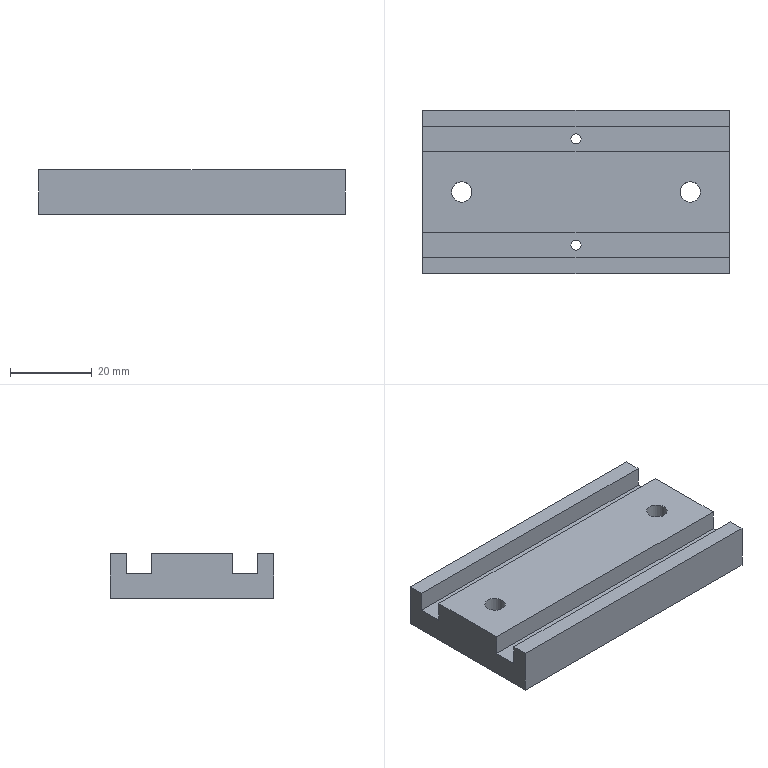Component | NX | MIDDLE_SUPPORT_PLATFORM_2 | 1 solid | 22 faces | volume 28003 mm3 | plane 14 | cylinder 4 | cone 4 | commonest cylinder face diameters 5 x2 2.5 x2